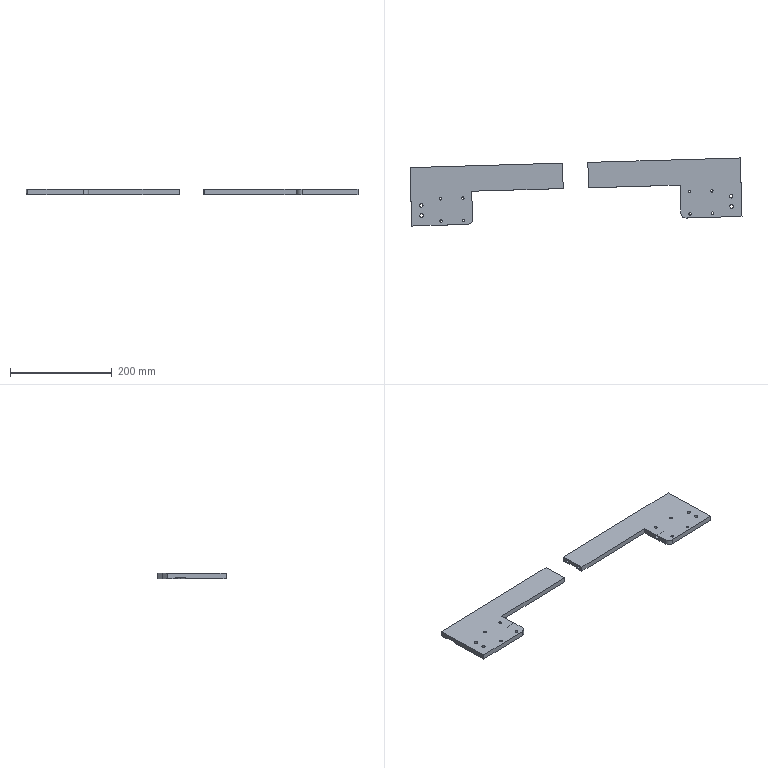Component | SolidWorks | ClampingCylinderMountingPlate-1 | 2 solids | 74 faces | volume 425299 mm3 | cylinder 38 | plane 24 | cone 12 | commonest cylinder face diameters 5 x24 6.8 x8 8.002 x4 20 x2 | material 6063